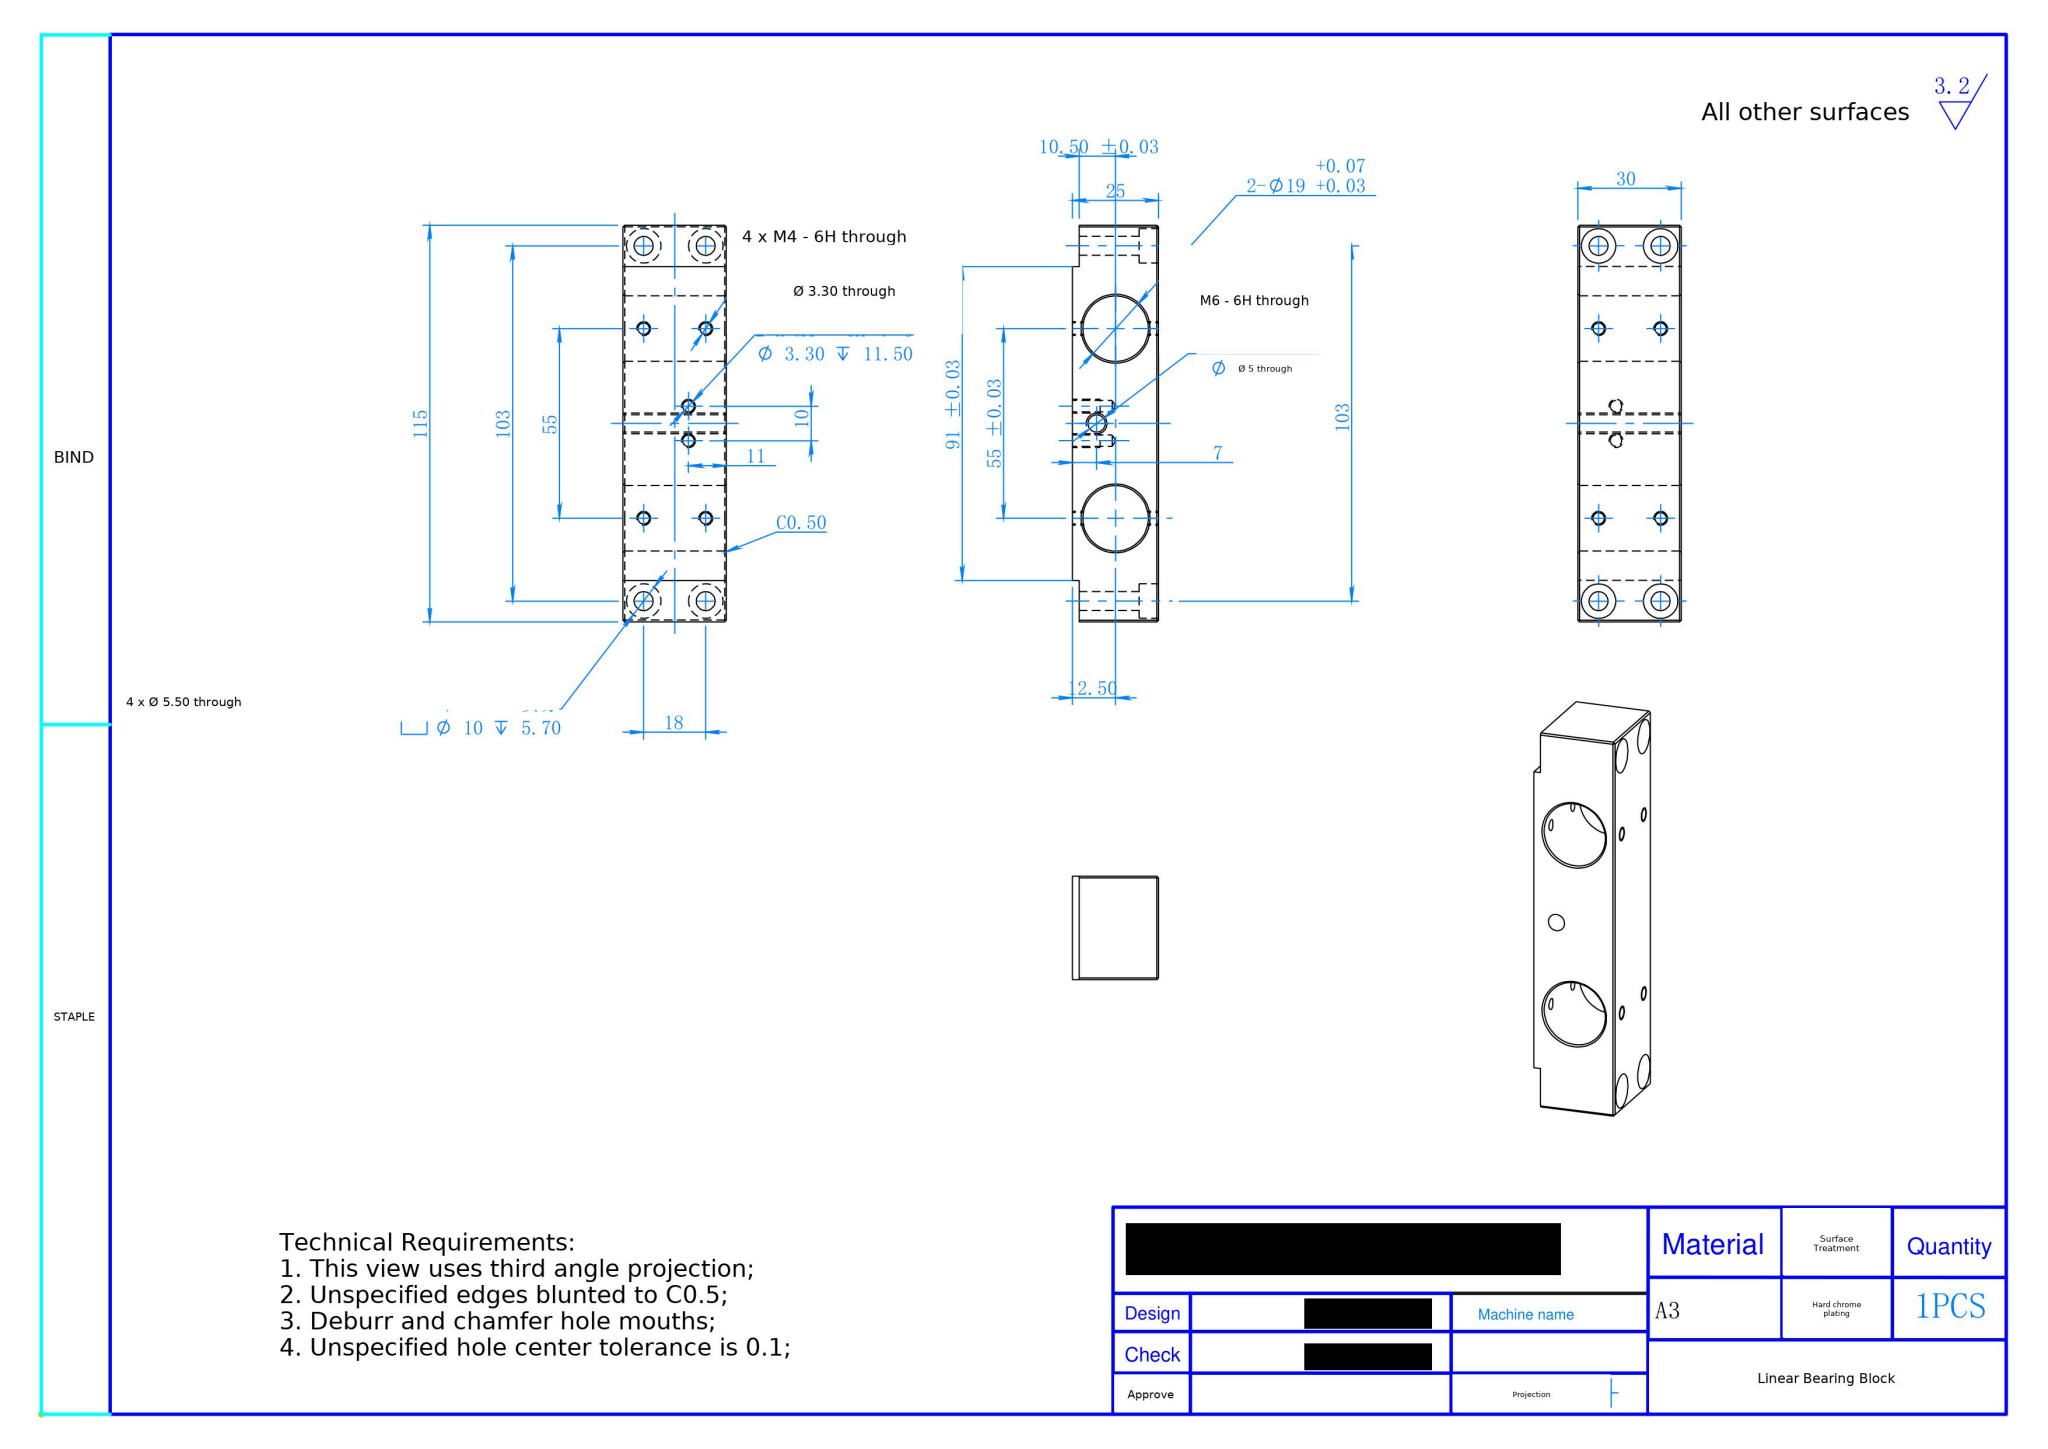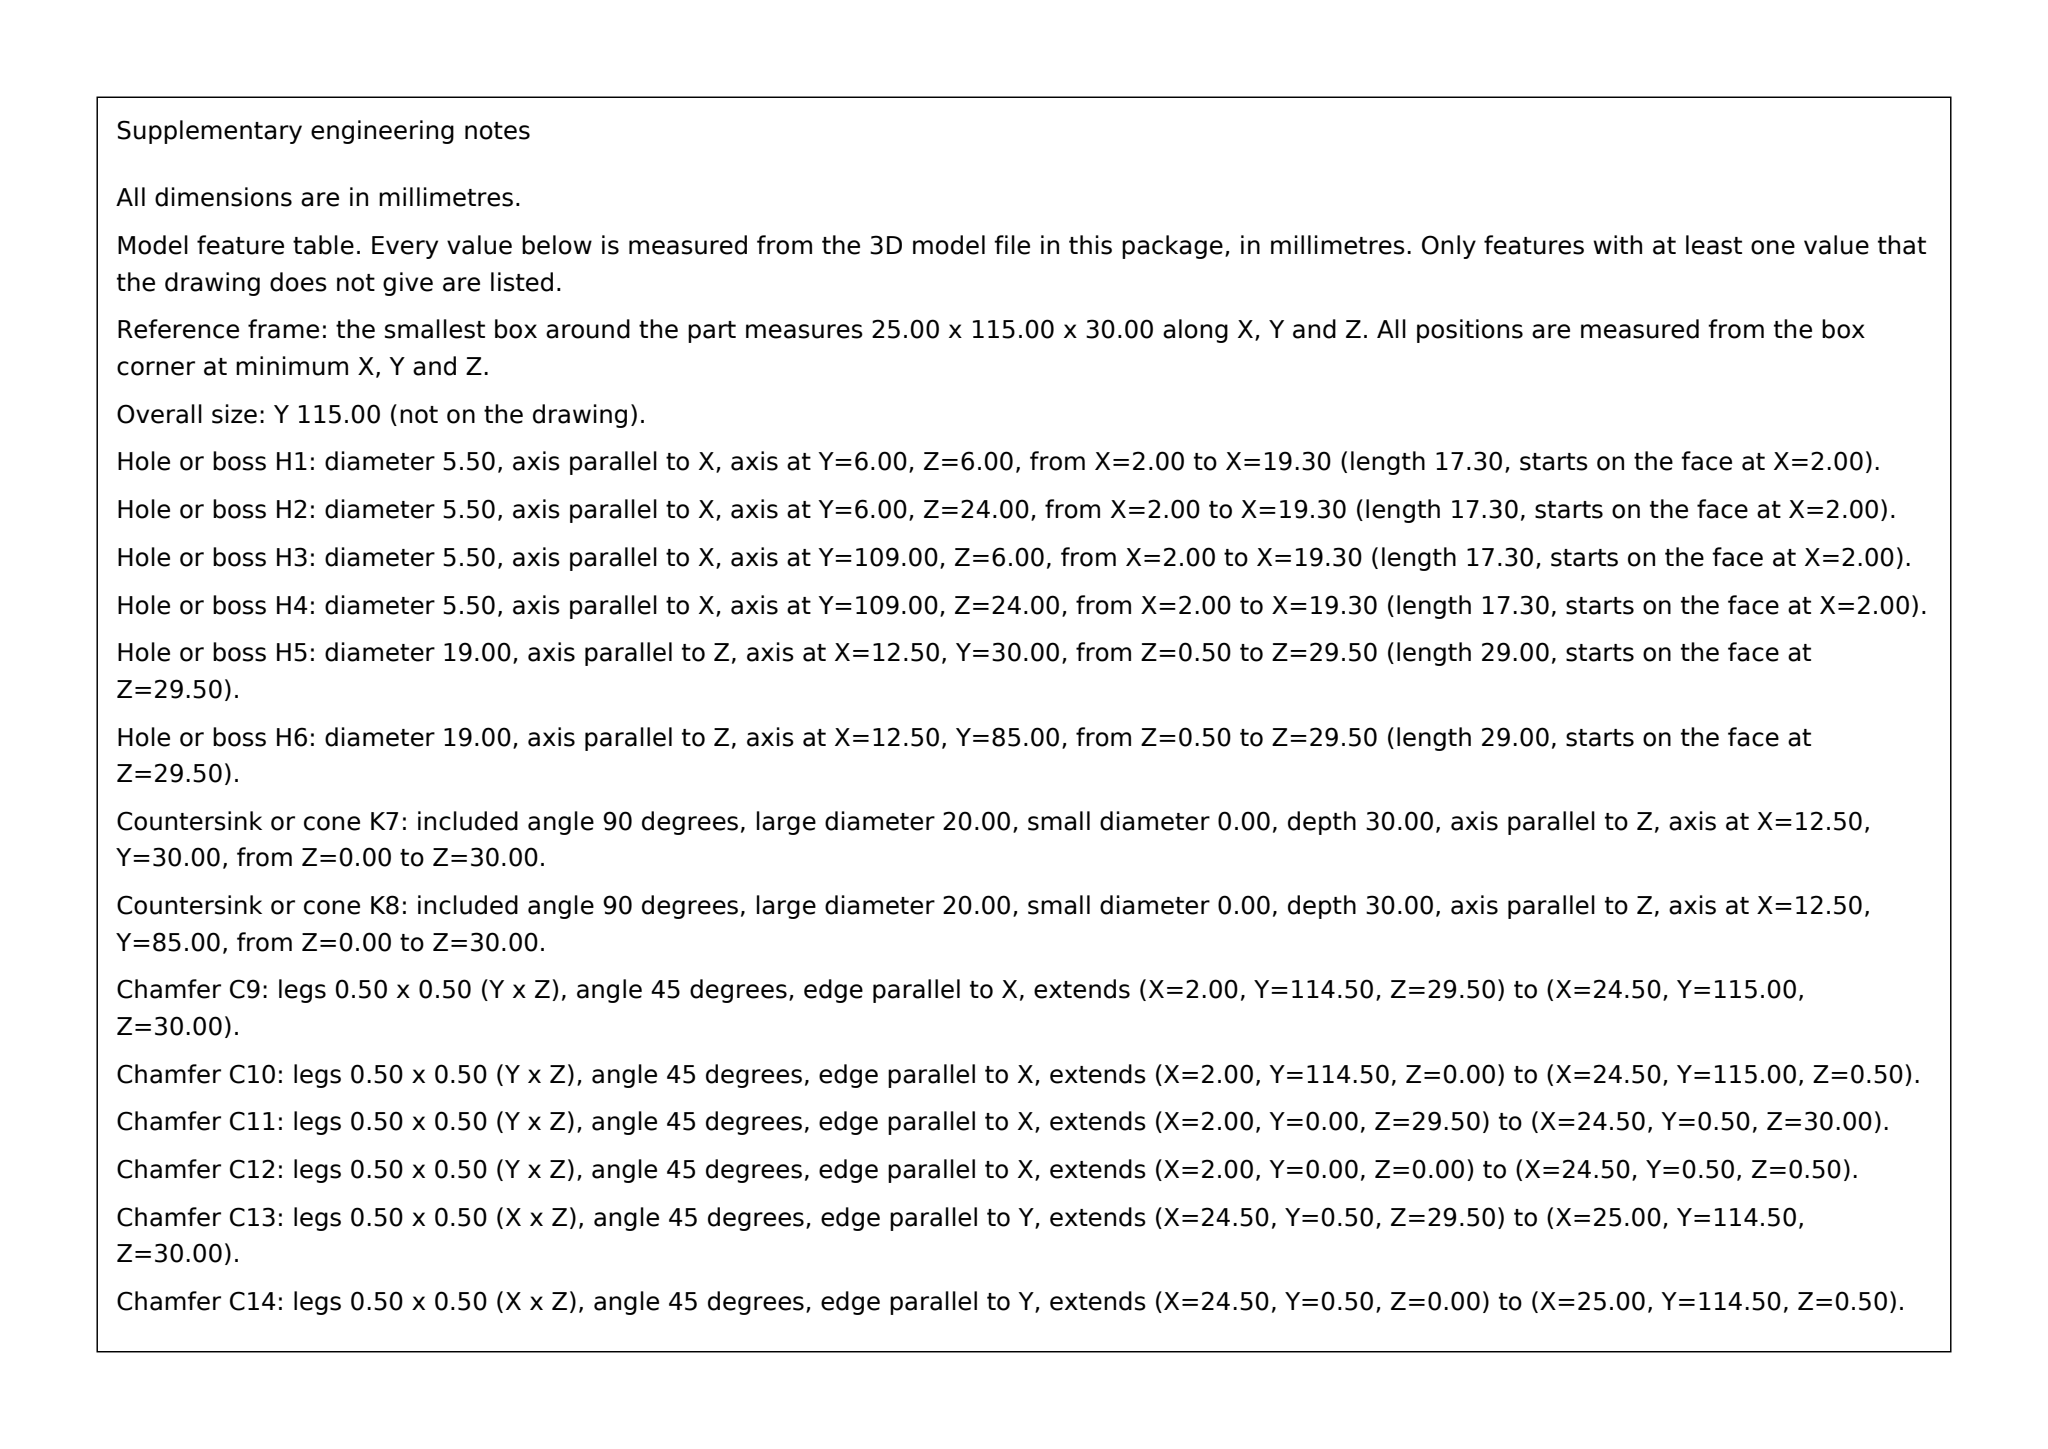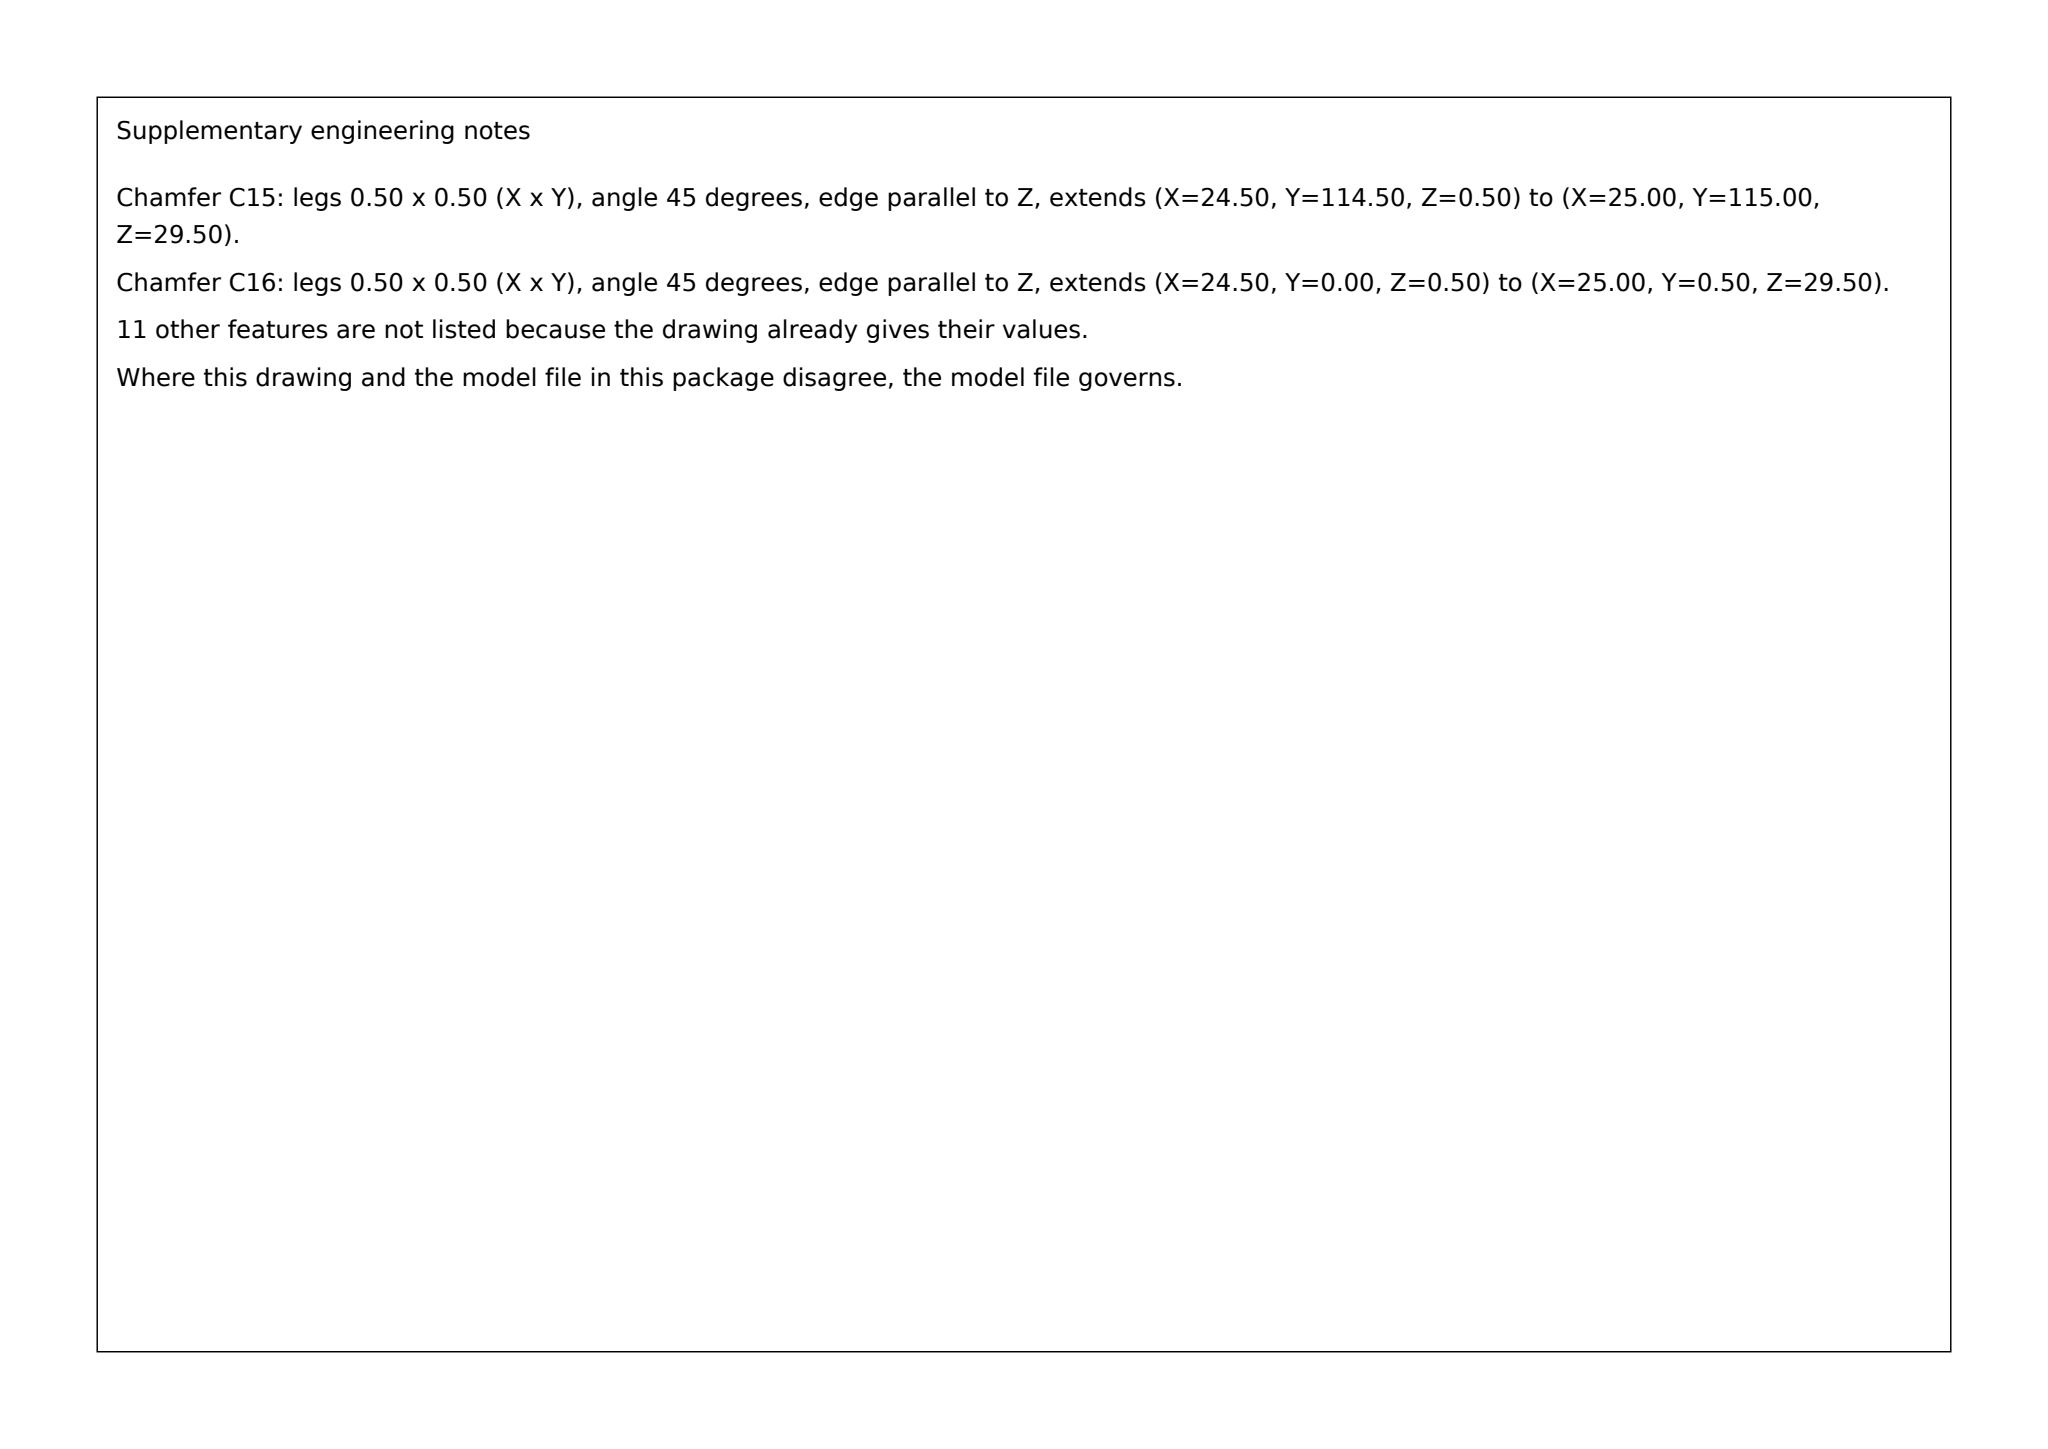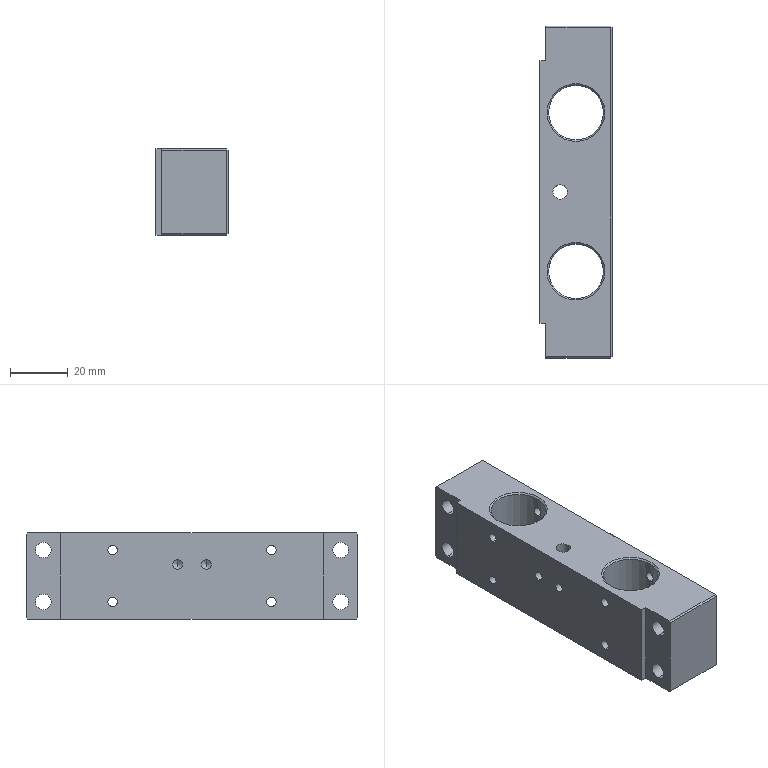Part | SolidWorks | mm | material A3 | 1 solid | 80 faces | box 25 x 115 x 30 mm | volume 63287 mm3 | cylinder 42 | plane 26 | cone 12 | commonest cylinder face diameters 3.3 x20 10 x8 5.5 x8 19 x4 5 x2
build123d program:
from build123d import *

# Parameters (mm, degrees)
SKETCH1_W                                         = 25
SKETCH1_H                                         = 115
SKETCH1_R                                         = 9.5
BOSS_EXTRUDE1_DEPTH                               = 30
M6_TAPPED_HOLE1_D                                 = 5
CHAMFER1_SIZE                                     = 0.5
HOLE_SIZE_ACCORDING_TO_HEX_SOCKET_HEA_D           = 5.5
HOLE_SIZE_ACCORDING_TO_HEX_SOCKET_HEA_CBORE_D     = 10
HOLE_SIZE_ACCORDING_TO_HEX_SOCKET_HEA_CBORE_DEPTH = 5.7
CHAMFER2_SIZE                                     = 0.5
M4_TAPPED_HOLE1_REACH                             = 93.793
M4_TAPPED_HOLE1_BORE_R                            = 1.65
SKETCH19_W                                        = 30
SKETCH19_H                                        = 12
CUT_EXTRUDE1_DEPTH                                = 2
M4_TAPPED_HOLE2_D                                 = 3.3
M4_TAPPED_HOLE2_DEPTH                             = 11.5
M4_TAPPED_HOLE2_TIP                               = 0.9914


with BuildPart() as part:
    # Sketch1 → Boss-Extrude1 (new body)
    with BuildSketch(Plane.XY):
        with Locations((12.5, 57.5)):
            Rectangle(SKETCH1_W, SKETCH1_H)
        with Locations((12.5, 85)):
            Circle(SKETCH1_R, mode=Mode.SUBTRACT)
        with Locations(Location((12.5, 30, 0), (0, 0, 180))):
            Circle(SKETCH1_R, mode=Mode.SUBTRACT)
    extrude(amount=BOSS_EXTRUDE1_DEPTH)

    # M6 Tapped Hole1 (through all)
    with Locations(Plane(origin=(7, 57.5, 0), x_dir=(-1, 0, 0), z_dir=(0, 0, -1))):
        with Locations((0, 0)):
            Hole(M6_TAPPED_HOLE1_D / 2)

    # Chamfer1
    chamfer1_edges = [part.edges().sort_by_distance(p)[0] for p in [
        (3, 85, 0),
        (3, 85, 30),
        (22, 30, 0),
        (22, 30, 30),
    ]]
    chamfer(chamfer1_edges, length=CHAMFER1_SIZE)

    # Hole Size _ according to_ Hex Socket Hea (through all)
    with Locations(Plane(origin=(25, 6, 24), x_dir=(0, 0, 1), z_dir=(1, 0, 0))):
        with Locations((0, 0), (-18, 0), (0, -103), (-18, -103)):
            CounterBoreHole(HOLE_SIZE_ACCORDING_TO_HEX_SOCKET_HEA_D / 2, HOLE_SIZE_ACCORDING_TO_HEX_SOCKET_HEA_CBORE_D / 2, HOLE_SIZE_ACCORDING_TO_HEX_SOCKET_HEA_CBORE_DEPTH)

    # Chamfer2
    chamfer2_edges = [part.edges().sort_by_distance(p)[0] for p in [
        (25, 57.5, 30),
        (12.5, 115, 30),
        (12.5, 115, 0),
        (25, 57.5, 0),
        (12.5, 0, 0),
        (12.5, 0, 30),
        (25, 115, 15),
        (25, 0, 15),
    ]]
    chamfer(chamfer2_edges, length=CHAMFER2_SIZE)

    # M4 Tapped Hole1 bore (on position points) → M4 Tapped Hole1 (cut, up to next)
    with BuildSketch(Plane(origin=(25, 30, 24), x_dir=(0, 0, 1), z_dir=(1, 0, 0)), mode=Mode.PRIVATE) as m4_tapped_hole1_sk1:
        Circle(M4_TAPPED_HOLE1_BORE_R)
    m4_tapped_hole1_tool1 = extrude(m4_tapped_hole1_sk1.sketch, amount=-M4_TAPPED_HOLE1_REACH, mode=Mode.PRIVATE) & part.part
    # M4 Tapped Hole1 bore (on position points) → M4 Tapped Hole1 (cut, up to next)
    with BuildSketch(Plane(origin=(25, 30, 24), x_dir=(0, 0, 1), z_dir=(1, 0, 0)), mode=Mode.PRIVATE) as m4_tapped_hole1_sk2:
        with Locations((-18, 0)):
            Circle(M4_TAPPED_HOLE1_BORE_R)
    m4_tapped_hole1_tool2 = extrude(m4_tapped_hole1_sk2.sketch, amount=-M4_TAPPED_HOLE1_REACH, mode=Mode.PRIVATE) & part.part
    # M4 Tapped Hole1 bore (on position points) → M4 Tapped Hole1 (cut, up to next)
    with BuildSketch(Plane(origin=(25, 30, 24), x_dir=(0, 0, 1), z_dir=(1, 0, 0)), mode=Mode.PRIVATE) as m4_tapped_hole1_sk3:
        with Locations((-18, -55)):
            Circle(M4_TAPPED_HOLE1_BORE_R)
    m4_tapped_hole1_tool3 = extrude(m4_tapped_hole1_sk3.sketch, amount=-M4_TAPPED_HOLE1_REACH, mode=Mode.PRIVATE) & part.part
    # M4 Tapped Hole1 bore (on position points) → M4 Tapped Hole1 (cut, up to next)
    with BuildSketch(Plane(origin=(25, 30, 24), x_dir=(0, 0, 1), z_dir=(1, 0, 0)), mode=Mode.PRIVATE) as m4_tapped_hole1_sk4:
        with Locations((0, -55)):
            Circle(M4_TAPPED_HOLE1_BORE_R)
    m4_tapped_hole1_tool4 = extrude(m4_tapped_hole1_sk4.sketch, amount=-M4_TAPPED_HOLE1_REACH, mode=Mode.PRIVATE) & part.part
    m4_tapped_hole1_1 = m4_tapped_hole1_tool1.solids().sort_by_distance((25, 30, 24))[0]
    add(m4_tapped_hole1_1, mode=Mode.SUBTRACT)
    m4_tapped_hole1_2 = m4_tapped_hole1_tool2.solids().sort_by_distance((25, 30, 6))[0]
    add(m4_tapped_hole1_2, mode=Mode.SUBTRACT)
    m4_tapped_hole1_3 = m4_tapped_hole1_tool3.solids().sort_by_distance((25, 85, 6))[0]
    add(m4_tapped_hole1_3, mode=Mode.SUBTRACT)
    m4_tapped_hole1_4 = m4_tapped_hole1_tool4.solids().sort_by_distance((25, 85, 24))[0]
    add(m4_tapped_hole1_4, mode=Mode.SUBTRACT)
    m4_tapped_hole1 = m4_tapped_hole1_1 + m4_tapped_hole1_2 + m4_tapped_hole1_3 + m4_tapped_hole1_4  # M4 Tapped Hole1 as one shape, for the pattern or mirror that repeats it

    # Mirror3: M4 Tapped Hole1 across plane
    add(m4_tapped_hole1.mirror(Plane(origin=(12.5, 0, 0), x_dir=(0, 0, 1), z_dir=(1, 0, 0))), mode=Mode.SUBTRACT)

    # Sketch19 → Cut-Extrude1 (cut)
    with BuildSketch(Plane.ZY):
        with Locations((15, 6)):
            Rectangle(SKETCH19_W, SKETCH19_H)
    cut_extrude1 = extrude(amount=-CUT_EXTRUDE1_DEPTH, mode=Mode.SUBTRACT)

    # Mirror4: Cut-Extrude1 across plane
    add(cut_extrude1.mirror(Plane(origin=(0, 57.5, 0), x_dir=(0, 0, 1), z_dir=(0, -1, 0))), mode=Mode.SUBTRACT)

    # M4 Tapped Hole2
    with Locations(Plane(origin=(0, -111.285, -74.478), x_dir=(0, 0, 1), z_dir=(-1, 0, 0))):
        with Locations((93.478, 173.785), (93.478, 163.785)):
            Hole(M4_TAPPED_HOLE2_D / 2, depth=M4_TAPPED_HOLE2_DEPTH)
            with Locations((0, 0, -(M4_TAPPED_HOLE2_DEPTH + M4_TAPPED_HOLE2_TIP / 2))):  # 118° drill point
                Cone(0, M4_TAPPED_HOLE2_D / 2, M4_TAPPED_HOLE2_TIP, mode=Mode.SUBTRACT)


solid = part.part